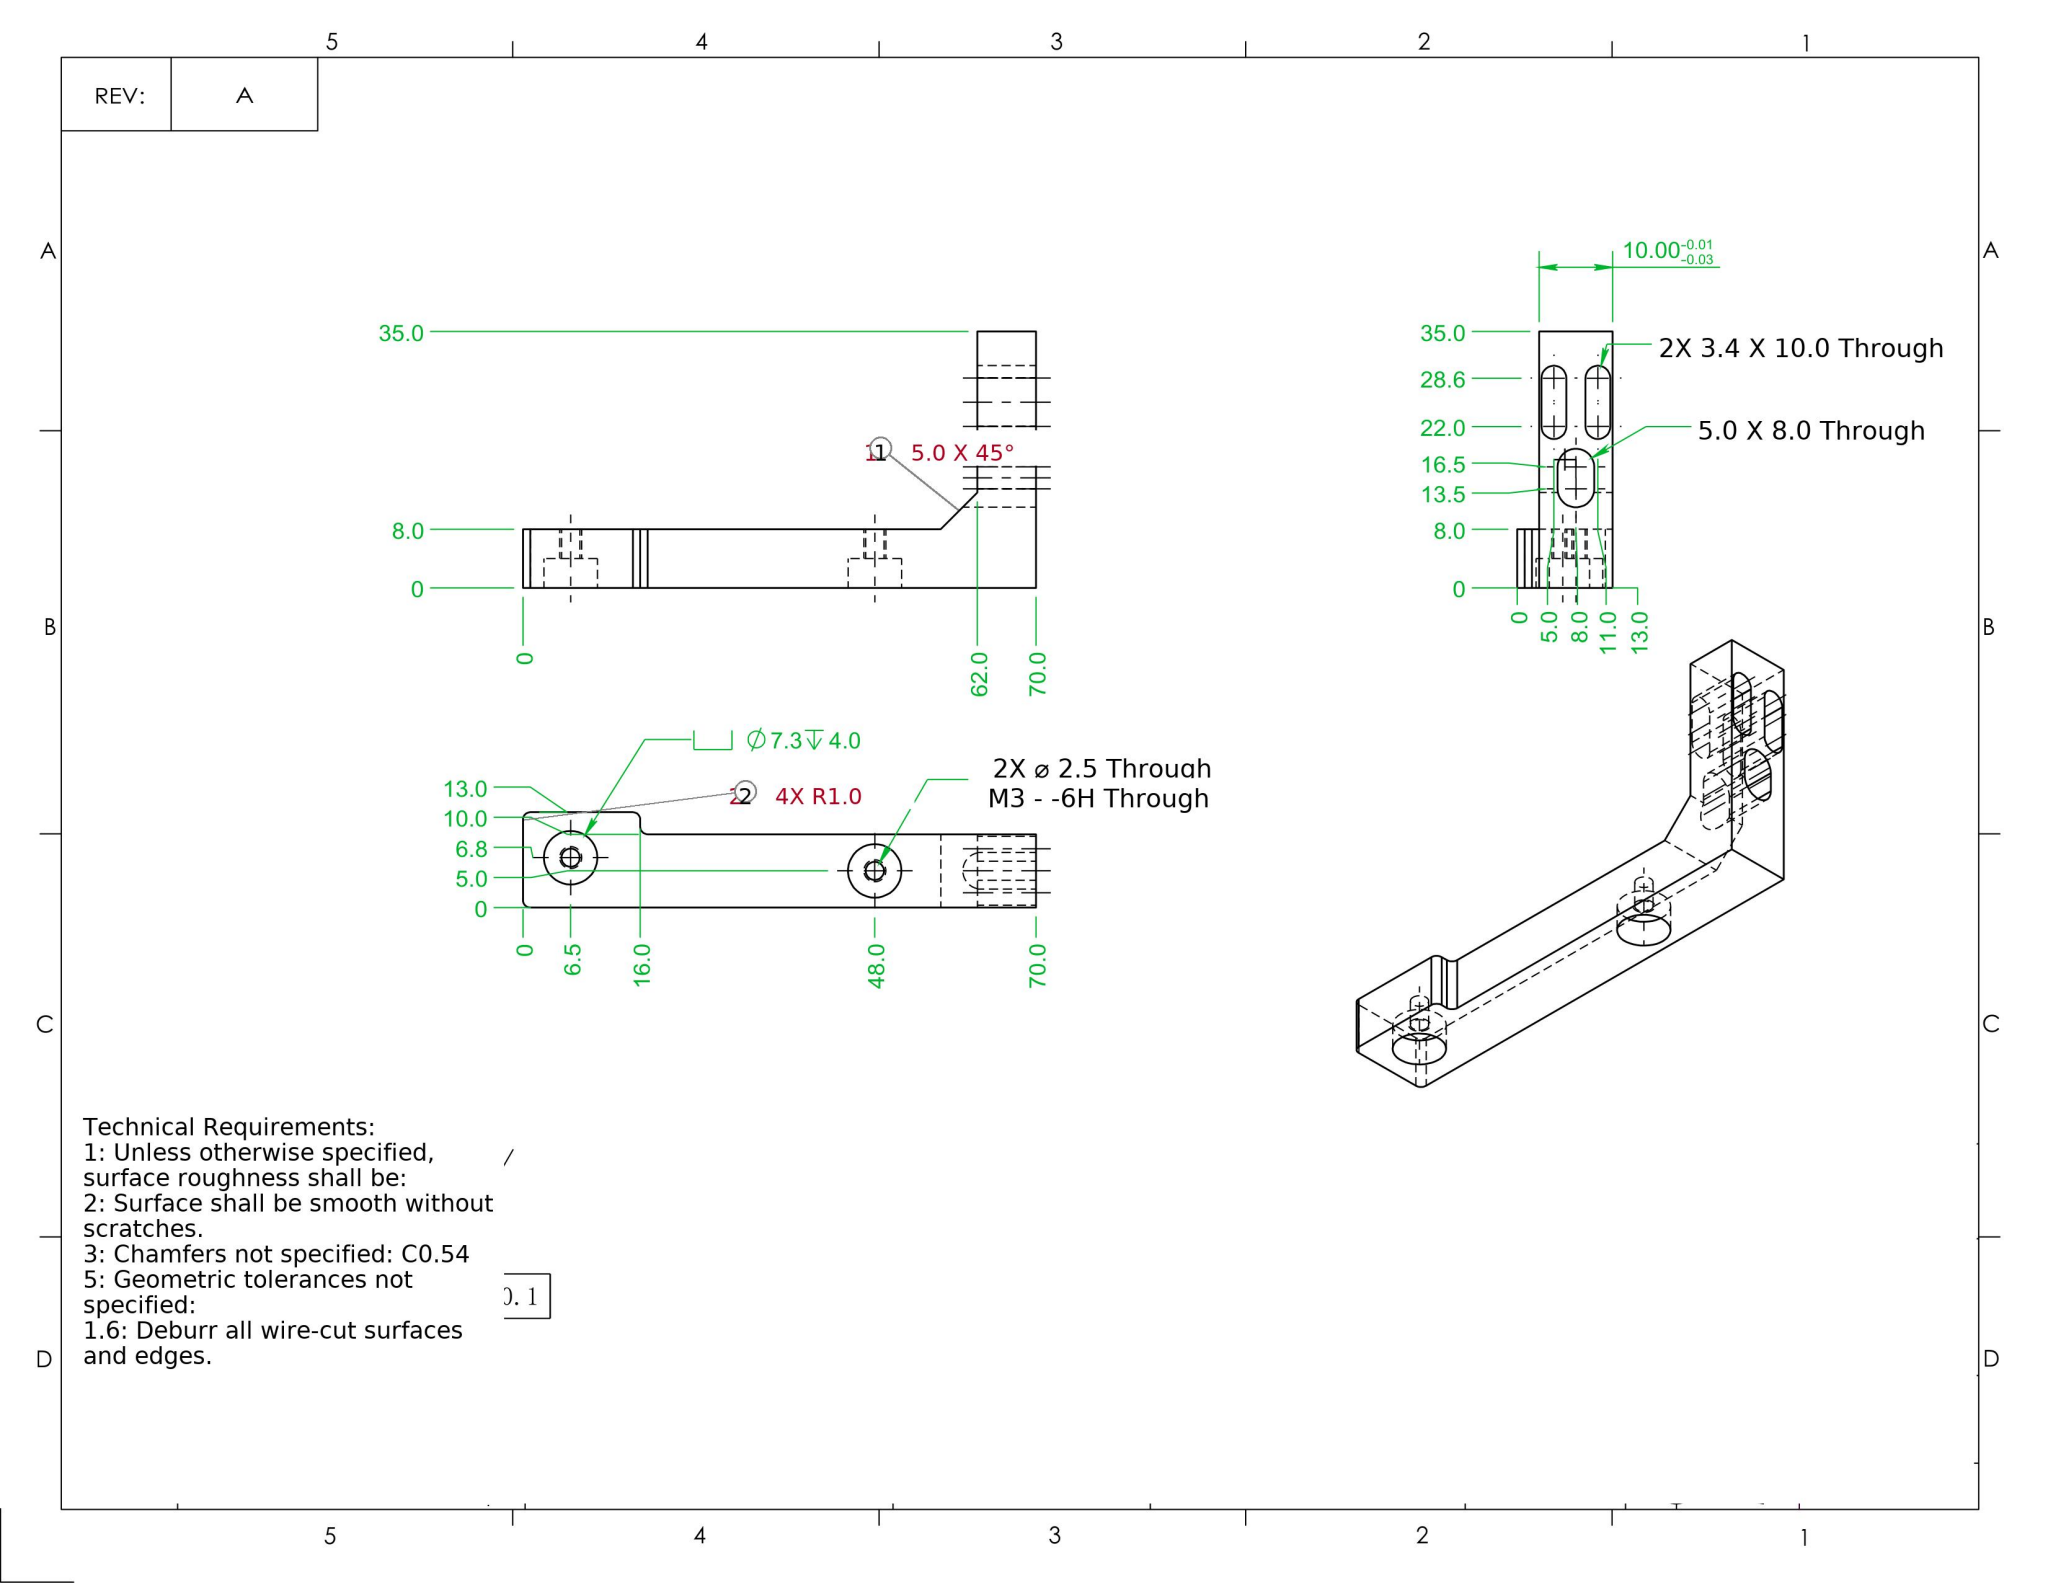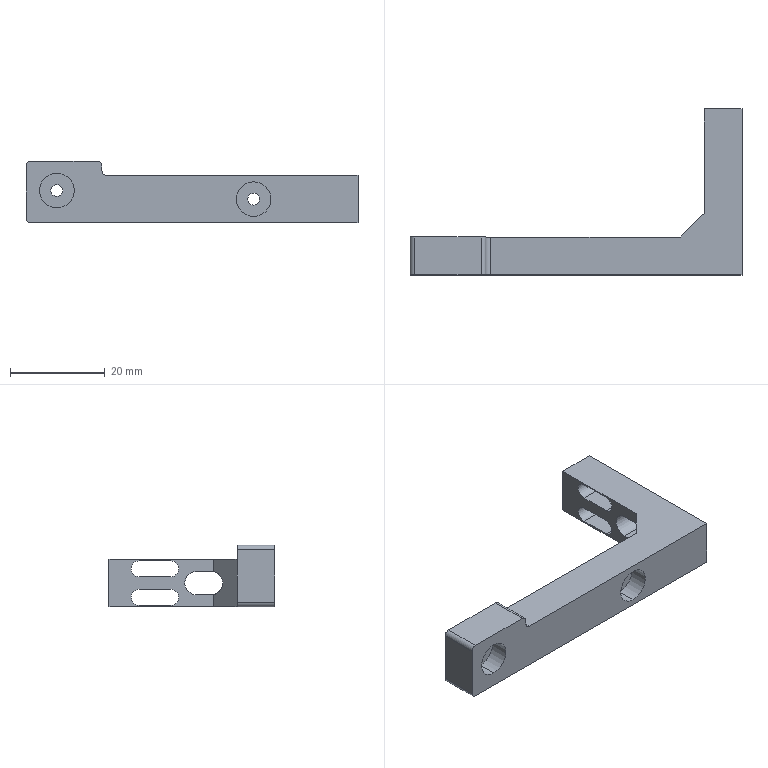Part | SolidWorks | mm | 1 solid | 37 faces | box 70 x 35 x 13 mm | volume 7104 mm3 | plane 19 | cylinder 18 | commonest cylinder face diameters 2.5 x4 7.3 x4 2 x4 3.4 x4 5 x2